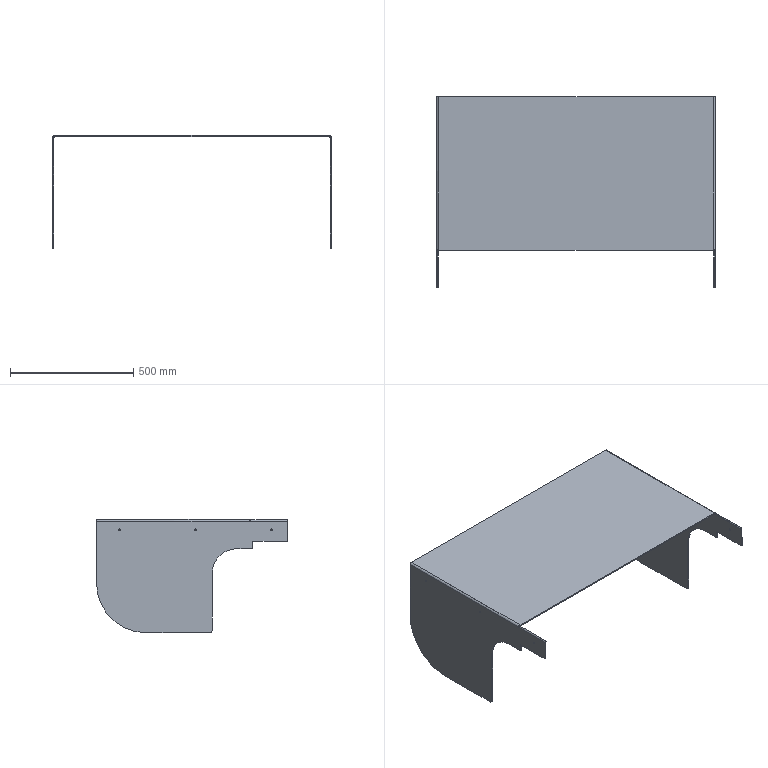Component | SolidWorks | FrontGuard-1 | 1 solid | 54 faces | volume 5908647 mm3 | plane 30 | cylinder 22 | spline 2 | commonest cylinder face diameters 7.2 x12 6 x2 16 x2 200 x2 20 x2 400 x2 | material Q235